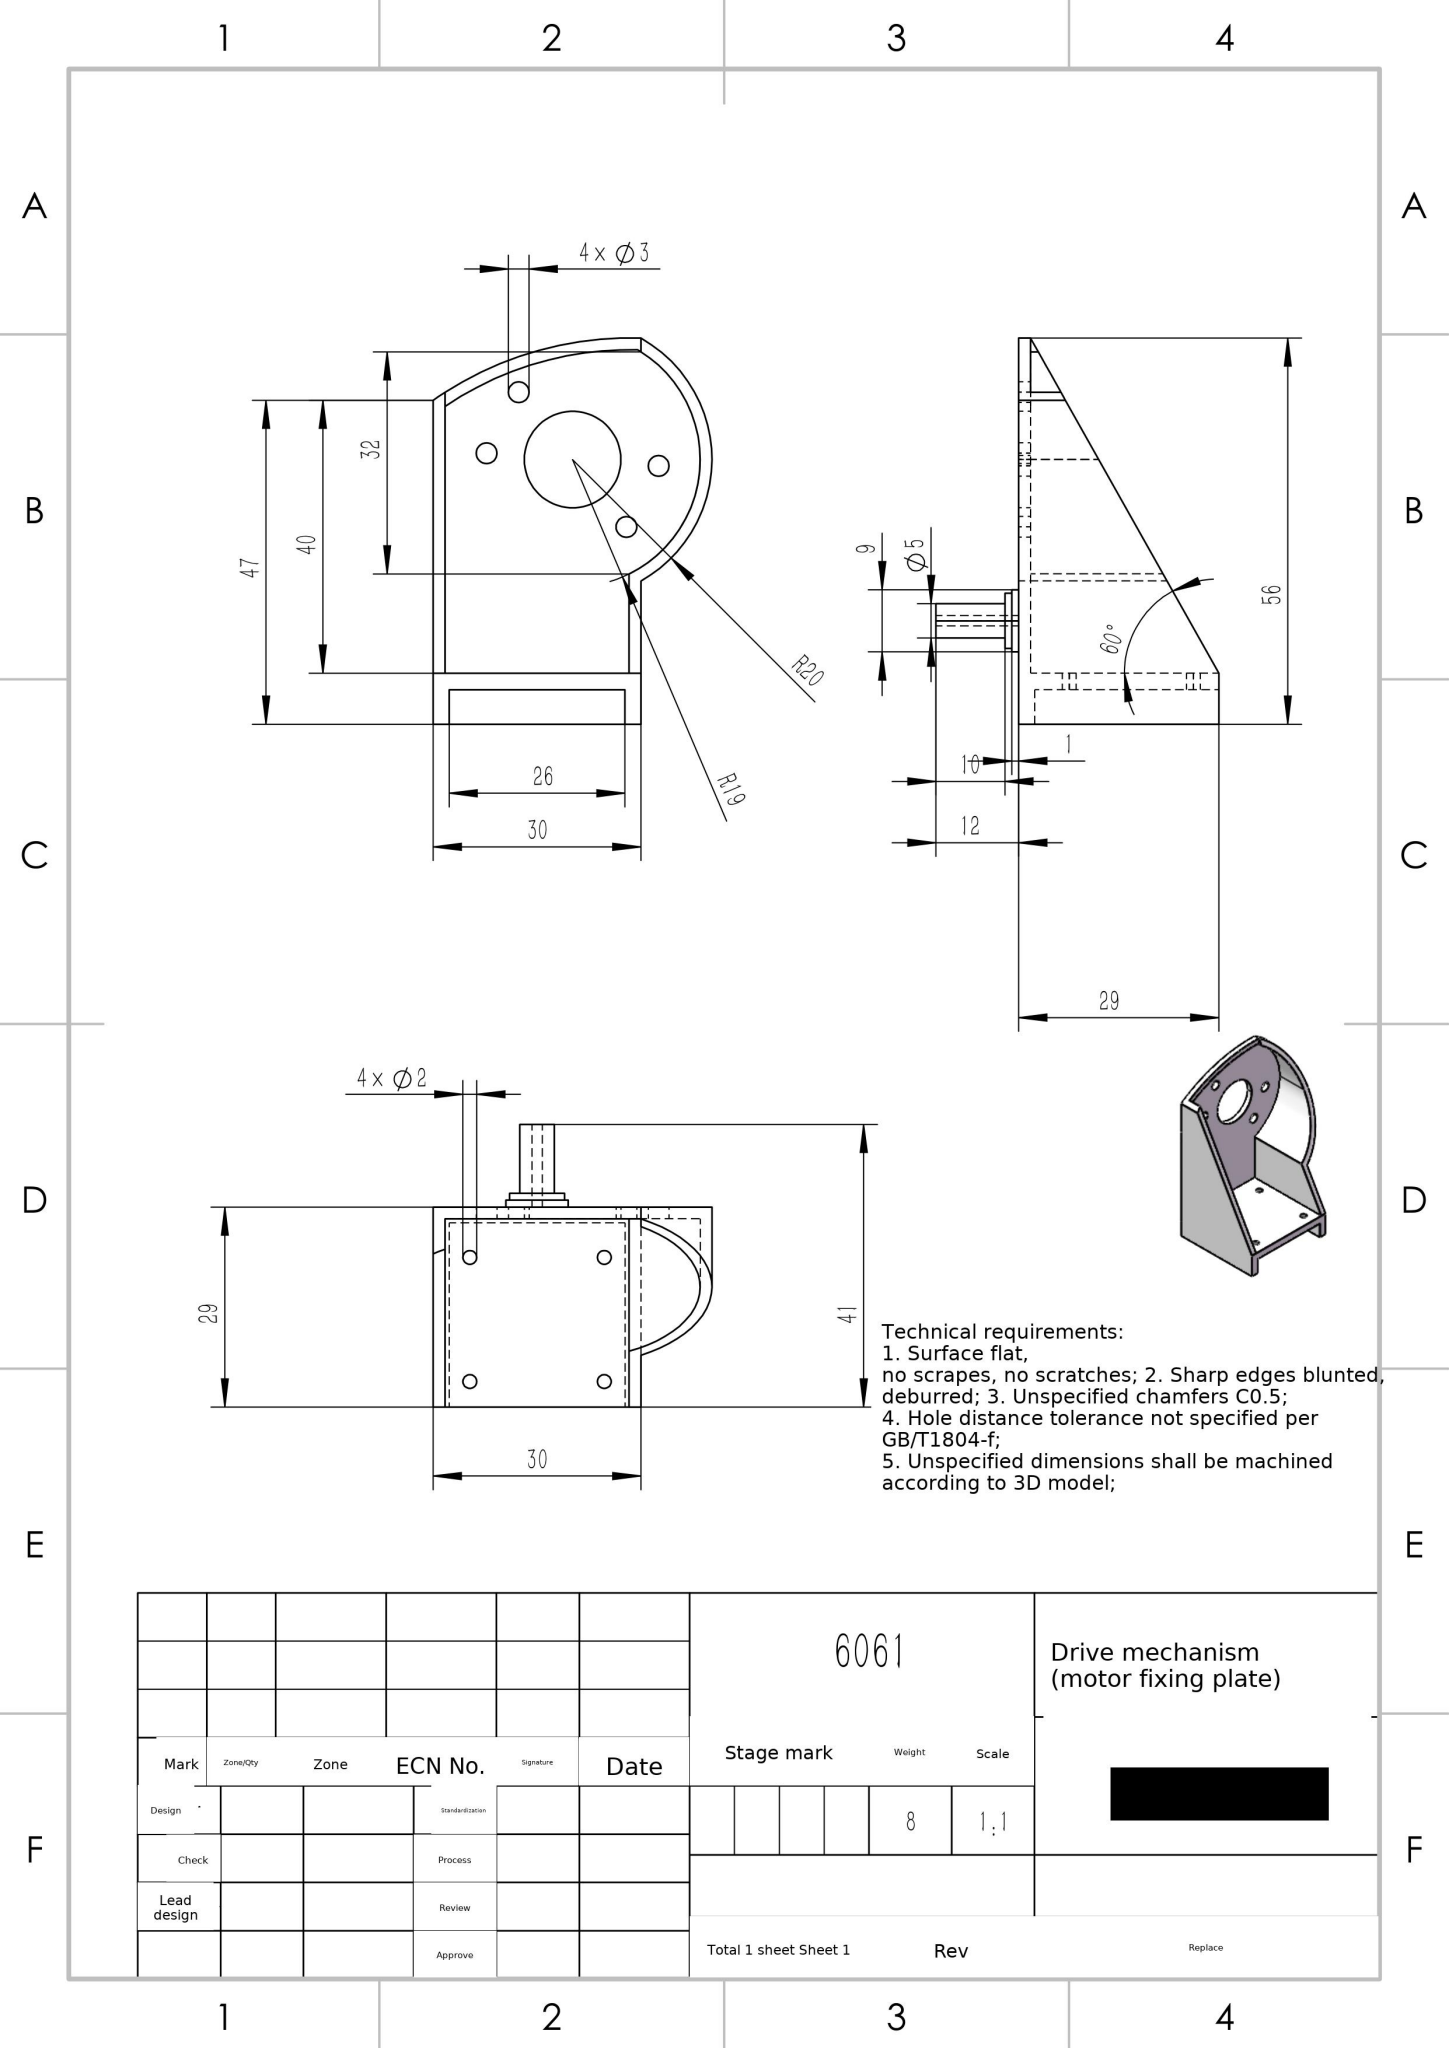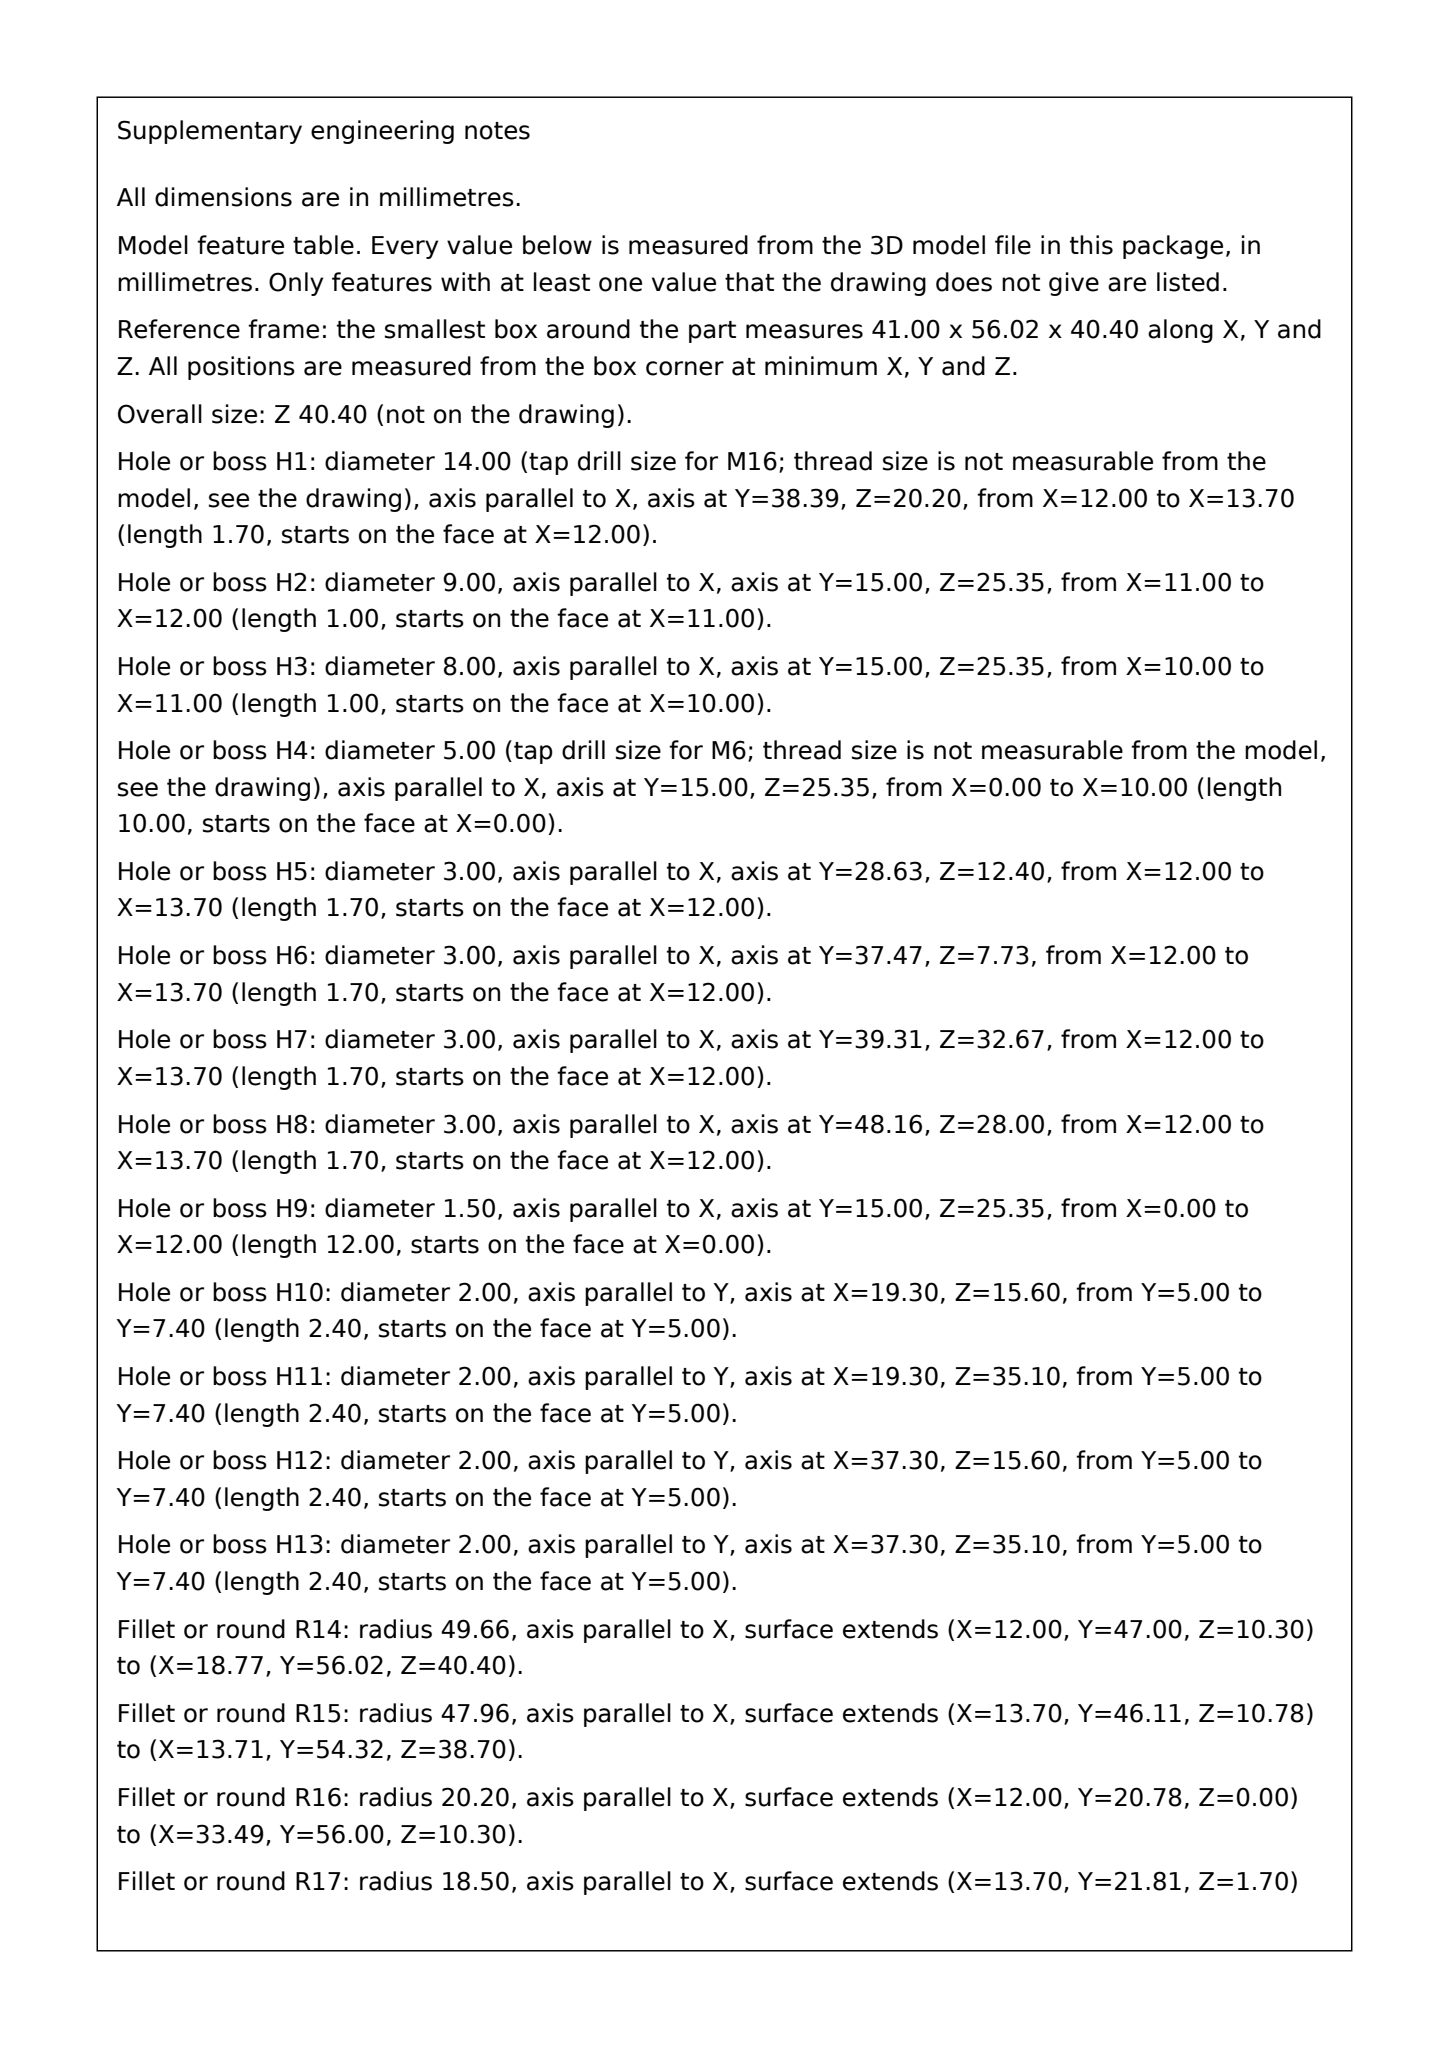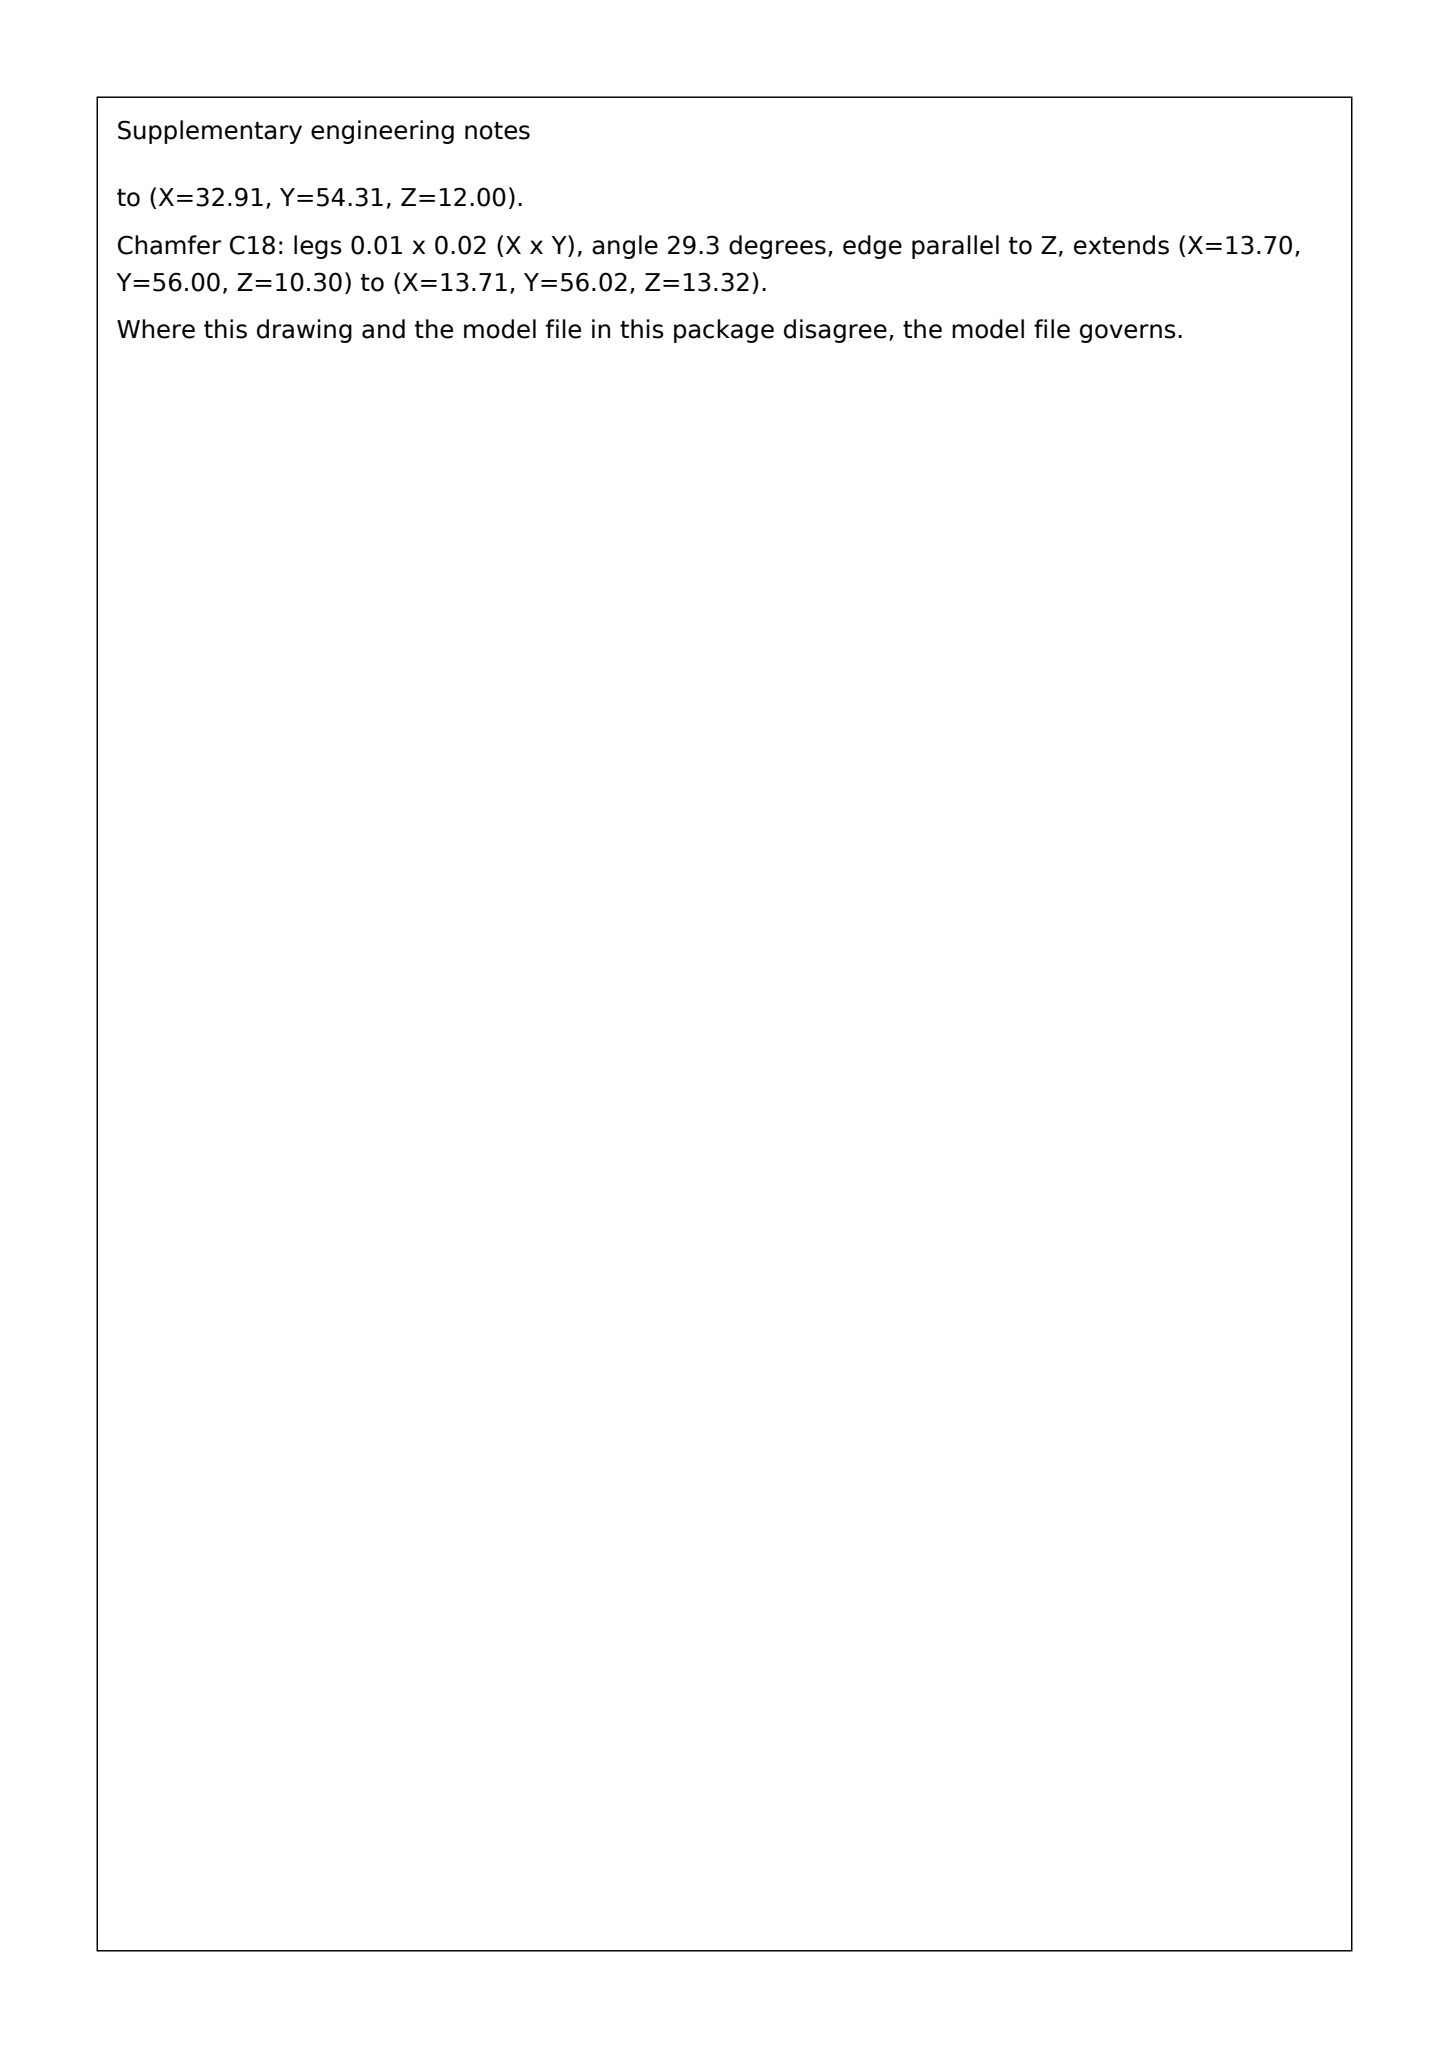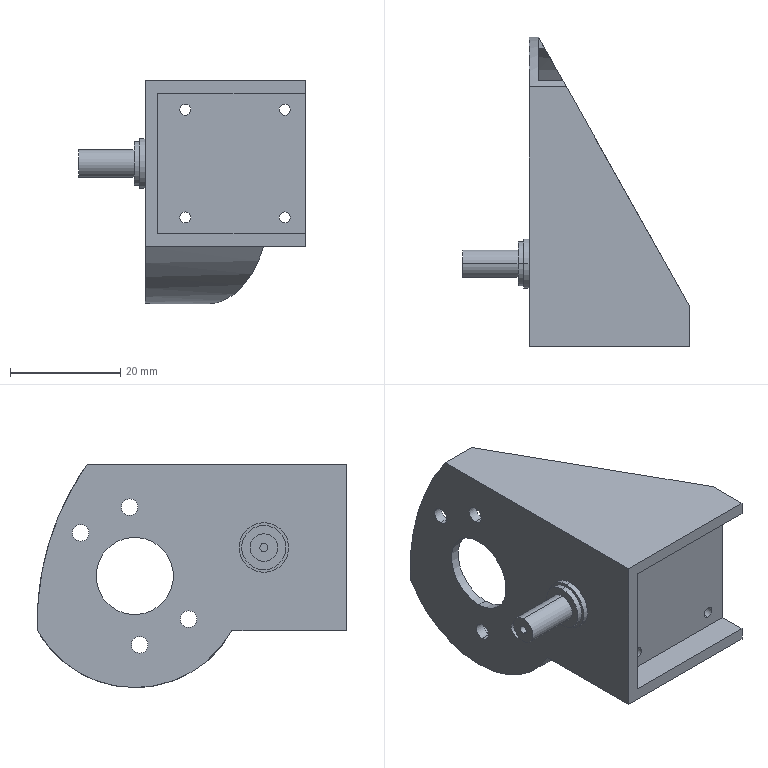Part | SolidWorks | mm | material 6061 | 1 solid | 54 faces | box 41 x 56.02 x 40.4 mm | volume 8142 mm3 | cylinder 32 | plane 22 | commonest cylinder face diameters 2 x8 3 x8 1.5 x2 5 x2 8 x2 9 x2 14 x2 40.4 x2